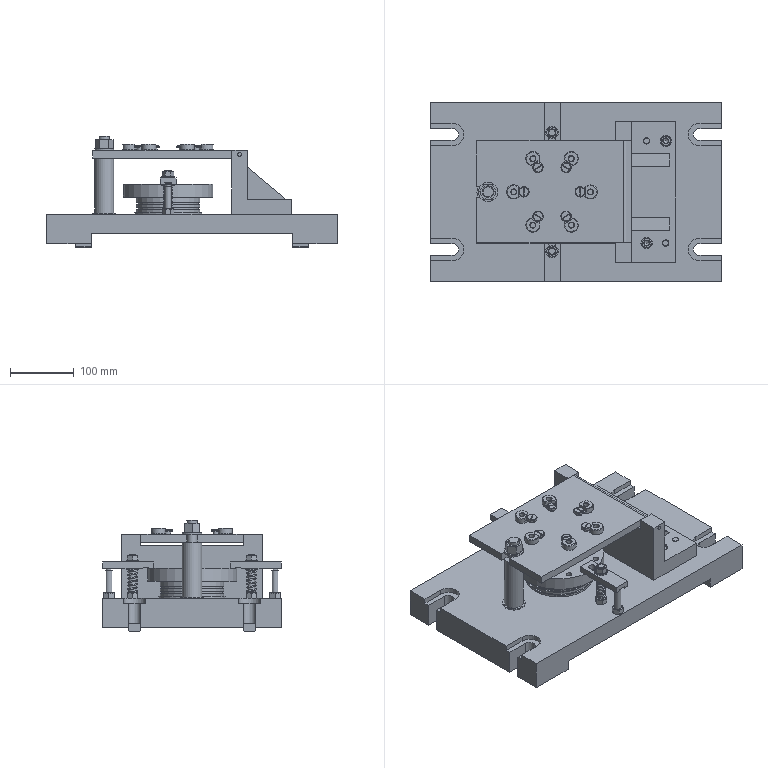Assembly | NX | mm | 51 component files | 51 solids | 825 faces | box 455 x 280 x 174 mm | volume 6250410 mm3 | plane 430 | cone 208 | cylinder 163 | torus 12 | spline 10 | sphere 2 | commonest cylinder face diameters 10 x26 6 x20 11 x16 12 x13 8.5 x12 16 x12 22 x6 5 x6
Bill of materials:
GB-T6170_F-2000,M16x2 | 1 |  | Hexagonal prism with a plain central through bore; corners chamfered (curved arc edges) on both end faces and a small countersink at the bore entry. Hex-nut-like shape, relatively tall for its width.
unnamed part 1 | 1 |  | Long, thin, solid cylindrical rod with flat ends and constant diameter.
unnamed part 2 | 2 |  | Cylindrical pin with a short, larger-diameter domed head; a narrow neck/groove sits just below the head, followed by a long plain shank with a flat end.
unnamed part 3 | 2 |  | Plain solid cylinder (rod section) with flat ends and no visible holes or steps.
GB-T95-2002,M10 | 4 |  | Plain Washer, GB-T 95-2002,M10
unnamed part 4 | 6 |  | Slotted-head shouldered pin/screw shape: a wide, thin head with chamfered top edge and a straight slot across the top, a shorter shoulder of medium diameter, a narrow neck, then a cylindrical shank.
GB-T6170_F-2000,M10x1.5 | 6 |  | Hexagonal prism with a plain central through bore, chamfered corners on both ends and a countersunk bore entry. Hex-nut-like shape, slightly thinner than unnamed part.
GB-T70.1-2000,M10x25 | 2 |  | Hexagon Socket Head Cap Screw, GB-T 70.1-2000,M10x25
GB-T119.1-2000,10x40 | 2 |  | Parallel Pin, GB-T 119.1-2000,10x40
unnamed part 5 | 4 |  | Rectangular block with one plain round through hole at the center of its large face; the four edges running along the long axis are chamfered.
unnamed part 6 | 1 |  | Solid stepped cylindrical shaft: a larger-diameter central section with smaller coaxial cylindrical journals extending from both ends.
unnamed part 7 | 6 |  | Flanged cylindrical bushing: a wide, short head with chamfered edges and a plain central through bore, over a smaller cylindrical spigot. One side of the head has a partial-depth flat/stepped cut, and the bore entry has a small chamfer.
GB-T70.1-2000,M6x10 | 4 |  | Hexagon Socket Head Cap Screw, GB-T 70.1-2000,M6x10
unnamed part 8 | 1 |  | Circular flange disk with six small through holes evenly spaced on a bolt circle and a central through bore with a shallow annular recess around it on the top face; a smaller-diameter cylindrical boss below has several circumferential grooves.
unnamed part 9 | 1 |  | Solid stepped cylindrical plug: a wider chamfered head, a short reduced-diameter undercut/neck, then a cylindrical body with chamfered edges and a flat end.
unnamed part 10 | 2 |  | Helical coil spring of round wire, constant coil diameter and pitch, with closed end coils that appear ground flat at both ends.
unnamed part 11 | 1 |  | L-shaped bracket: a rectangular base plate with an upright wall along one long edge, two triangular gussets joining wall and base, and raised blocks at both ends of the wall top; the base has through holes at each end.
unnamed part 12 | 1 |  | Thin rectangular plate with one edge rolled into a hollow cylindrical curl. It has a symmetric pattern of large and small holes and an open-ended rounded slot in the opposite edge.
GB-T95-2002,M16 | 1 |  | Plain Washer, GB-T 95-2002,M16
unnamed part 13 | 1 |  | Rectangular base plate with four open-ended counterbored U-slots, two at each short end. The middle of the underside is relieved, leaving thicker pads at the ends. The top has a central round hole with a shallow circular raised face, a smaller hole with a ring around it, and several small holes.
unnamed part 14 | 2 |  | Rectangular block with a through obround (elongated) slot along its length. The underside has a shallow transverse groove with angled edges near one end.
Mates:
1. concentric | dowel_pin 1 edge | fixture_body 1 edge
2. fix | fixture_body 1 component
3. concentric | cylinder_head 1 edge | fixture_body 1 edge
4. touch align | clamping_plate 2 face | cylinder_head 1 face
5. distance | clamping_plate 2 face | cylinder_head 1 face
6. touch align | fixing_screw 2 face | clamping_plate 2 face
7. concentric | GB-T95-2002_M10 4 edge | clamping_plate 2 edge
8. concentric | GB-T6170_F-2000_M10x1_5 6 edge | GB-T95-2002_M10 4 edge
9. distance | clamping_plate 2 face | fixing_screw 2 face
10. touch align | support_screw 2 face | fixture_body 1 face
11. touch align | support_screw 2 face | clamping_plate 2 face
12. concentric | GB-T6170_F-2000_M10x1_5 5 edge | fixture_body 1 arc
13. concentric | GB-T6170_F-2000_M10x1_5 4 edge | fixture_body 1 arc
14. touch align | GB-T95-2002_M10 3 face | fixing_screw 2 face
15. touch align | clamping_plate 2 face | GB-T95-2002_M10 3 face
16. concentric | spring 2 edge | GB-T6170_F-2000_M10x1_5 5 edge
17. bond | cylinder_head 1 component | assembly component
18. bond | GB-T6170_F-2000_M10x1_5 4 component | assembly component
19. bond | fixing_screw 2 component | assembly component
20. bond | clamping_plate 2 component | assembly component
21. bond | support_screw 2 component | assembly component
22. bond | GB-T95-2002_M10 4 component | assembly component
23. bond | GB-T6170_F-2000_M10x1_5 6 component | assembly component
24. bond | GB-T6170_F-2000_M10x1_5 5 component | assembly component
25. bond | GB-T95-2002_M10 3 component | assembly component
26. bond | spring 2 component | assembly component
27. bond | GB-T6170_F-2000_M10x1_5 3 component | assembly component
28. bond | fixing_screw 1 component | assembly component
29. bond | clamping_plate 1 component | assembly component
30. bond | support_screw 1 component | assembly component
31. bond | GB-T95-2002_M10 2 component | assembly component
32. bond | GB-T6170_F-2000_M10x1_5 2 component | assembly component
33. bond | GB-T6170_F-2000_M10x1_5 1 component | assembly component
34. bond | GB-T95-2002_M10 1 component | assembly component
35. bond | spring 1 component | assembly component
36. circular | assembly datumaxis | assembly cartesiancoordinatesystem | assembly cartesiancoordinatesystem
37. circular | assembly datumaxis | assembly cartesiancoordinatesystem | assembly cartesiancoordinatesystem
38. circular | assembly datumaxis | assembly cartesiancoordinatesystem | assembly cartesiancoordinatesystem
39. circular | assembly datumaxis | assembly cartesiancoordinatesystem | assembly cartesiancoordinatesystem
40. circular | assembly datumaxis | assembly cartesiancoordinatesystem | assembly cartesiancoordinatesystem
41. circular | assembly datumaxis | assembly cartesiancoordinatesystem | assembly cartesiancoordinatesystem
42. circular | assembly datumaxis | assembly cartesiancoordinatesystem | assembly cartesiancoordinatesystem
43. circular | assembly datumaxis | assembly cartesiancoordinatesystem | assembly cartesiancoordinatesystem
44. circular | assembly datumaxis | assembly cartesiancoordinatesystem | assembly cartesiancoordinatesystem
45. touch align | angle_bracket 1 face | fixture_body 1 face
46. distance | angle_bracket 1 face | cylinder_head 1 face
47. center | angle_bracket 1 face | angle_bracket 1 face | fixture_body 1 face | fixture_body 1 face
48. concentric | drill_bush 6 edge | drill_template 1 edge
49. concentric | drill_bush_screw 6 edge | drill_template 1 arc
50. concentric | drill_template 1 edge | angle_bracket 1 edge
51. touch align | drill_bush 6 face | cylinder_head 1 face
52. bond | cylinder_head 1 component | assembly component
53. bond | drill_bush 6 component | assembly component
54. bond | drill_bush_screw 6 component | assembly component
55. bond | drill_bush 5 component | assembly component
56. bond | drill_bush_screw 5 component | assembly component
57. circular | assembly datumaxis | assembly cartesiancoordinatesystem | assembly cartesiancoordinatesystem | assembly cartesiancoordinatesystem | assembly cartesiancoordinatesystem | assembly cartesiancoordinatesystem | assembly cartesiancoordinatesystem
58. circular | assembly datumaxis | assembly cartesiancoordinatesystem | assembly cartesiancoordinatesystem | assembly cartesiancoordinatesystem | assembly cartesiancoordinatesystem | assembly cartesiancoordinatesystem | assembly cartesiancoordinatesystem
59. bond | drill_bush 4 component | assembly component
60. bond | drill_bush_screw 4 component | assembly component
61. bond | drill_bush 3 component | assembly component
62. bond | drill_bush_screw 3 component | assembly component
63. bond | drill_bush 2 component | assembly component
64. bond | drill_bush_screw 2 component | assembly component
65. bond | drill_bush 1 component | assembly component
66. bond | drill_bush_screw 1 component | assembly component
67. concentric | support_rod 1 edge | fixture_body 1 edge
68. concentric | GB-T95-2002_M16 1 edge | drill_template 1 edge
69. concentric | GB-T6170_F-2000_M16x2 1 edge | GB-T95-2002_M16 1 edge
70. concentric | hinge 1 edge | angle_bracket 1 edge
71. touch align | locating_key 4 face | fixture_body 1 face
72. touch align | locating_key 4 face | fixture_body 1 face
73. touch align | locating_key 4 face | fixture_body 1 face
74. bond | fixture_body 1 component | assembly component
75. bond | fixture_body 1 component | assembly component
76. bond | locating_key 4 component | assembly component
77. bond | locating_key 3 component | assembly component
78. bond | locating_key 2 component | assembly component
79. bond | locating_key 1 component | assembly component
80. linear | assembly datumaxis | assembly datumaxis | assembly cartesiancoordinatesystem | assembly cartesiancoordinatesystem | assembly cartesiancoordinatesystem | assembly cartesiancoordinatesystem
81. bond | GB-T70_1-2000_M6x10 4 component | assembly component
82. bond | GB-T70_1-2000_M6x10 3 component | assembly component
83. bond | GB-T70_1-2000_M6x10 2 component | assembly component
84. bond | GB-T70_1-2000_M6x10 1 component | assembly component
85. linear | assembly datumaxis | assembly datumaxis | assembly cartesiancoordinatesystem | assembly cartesiancoordinatesystem | assembly cartesiancoordinatesystem | assembly cartesiancoordinatesystem
86. touch align | fixing_screw 2 face | fixture_body 1 face
87. touch align | support_screw 2 face | fixture_body 1 face